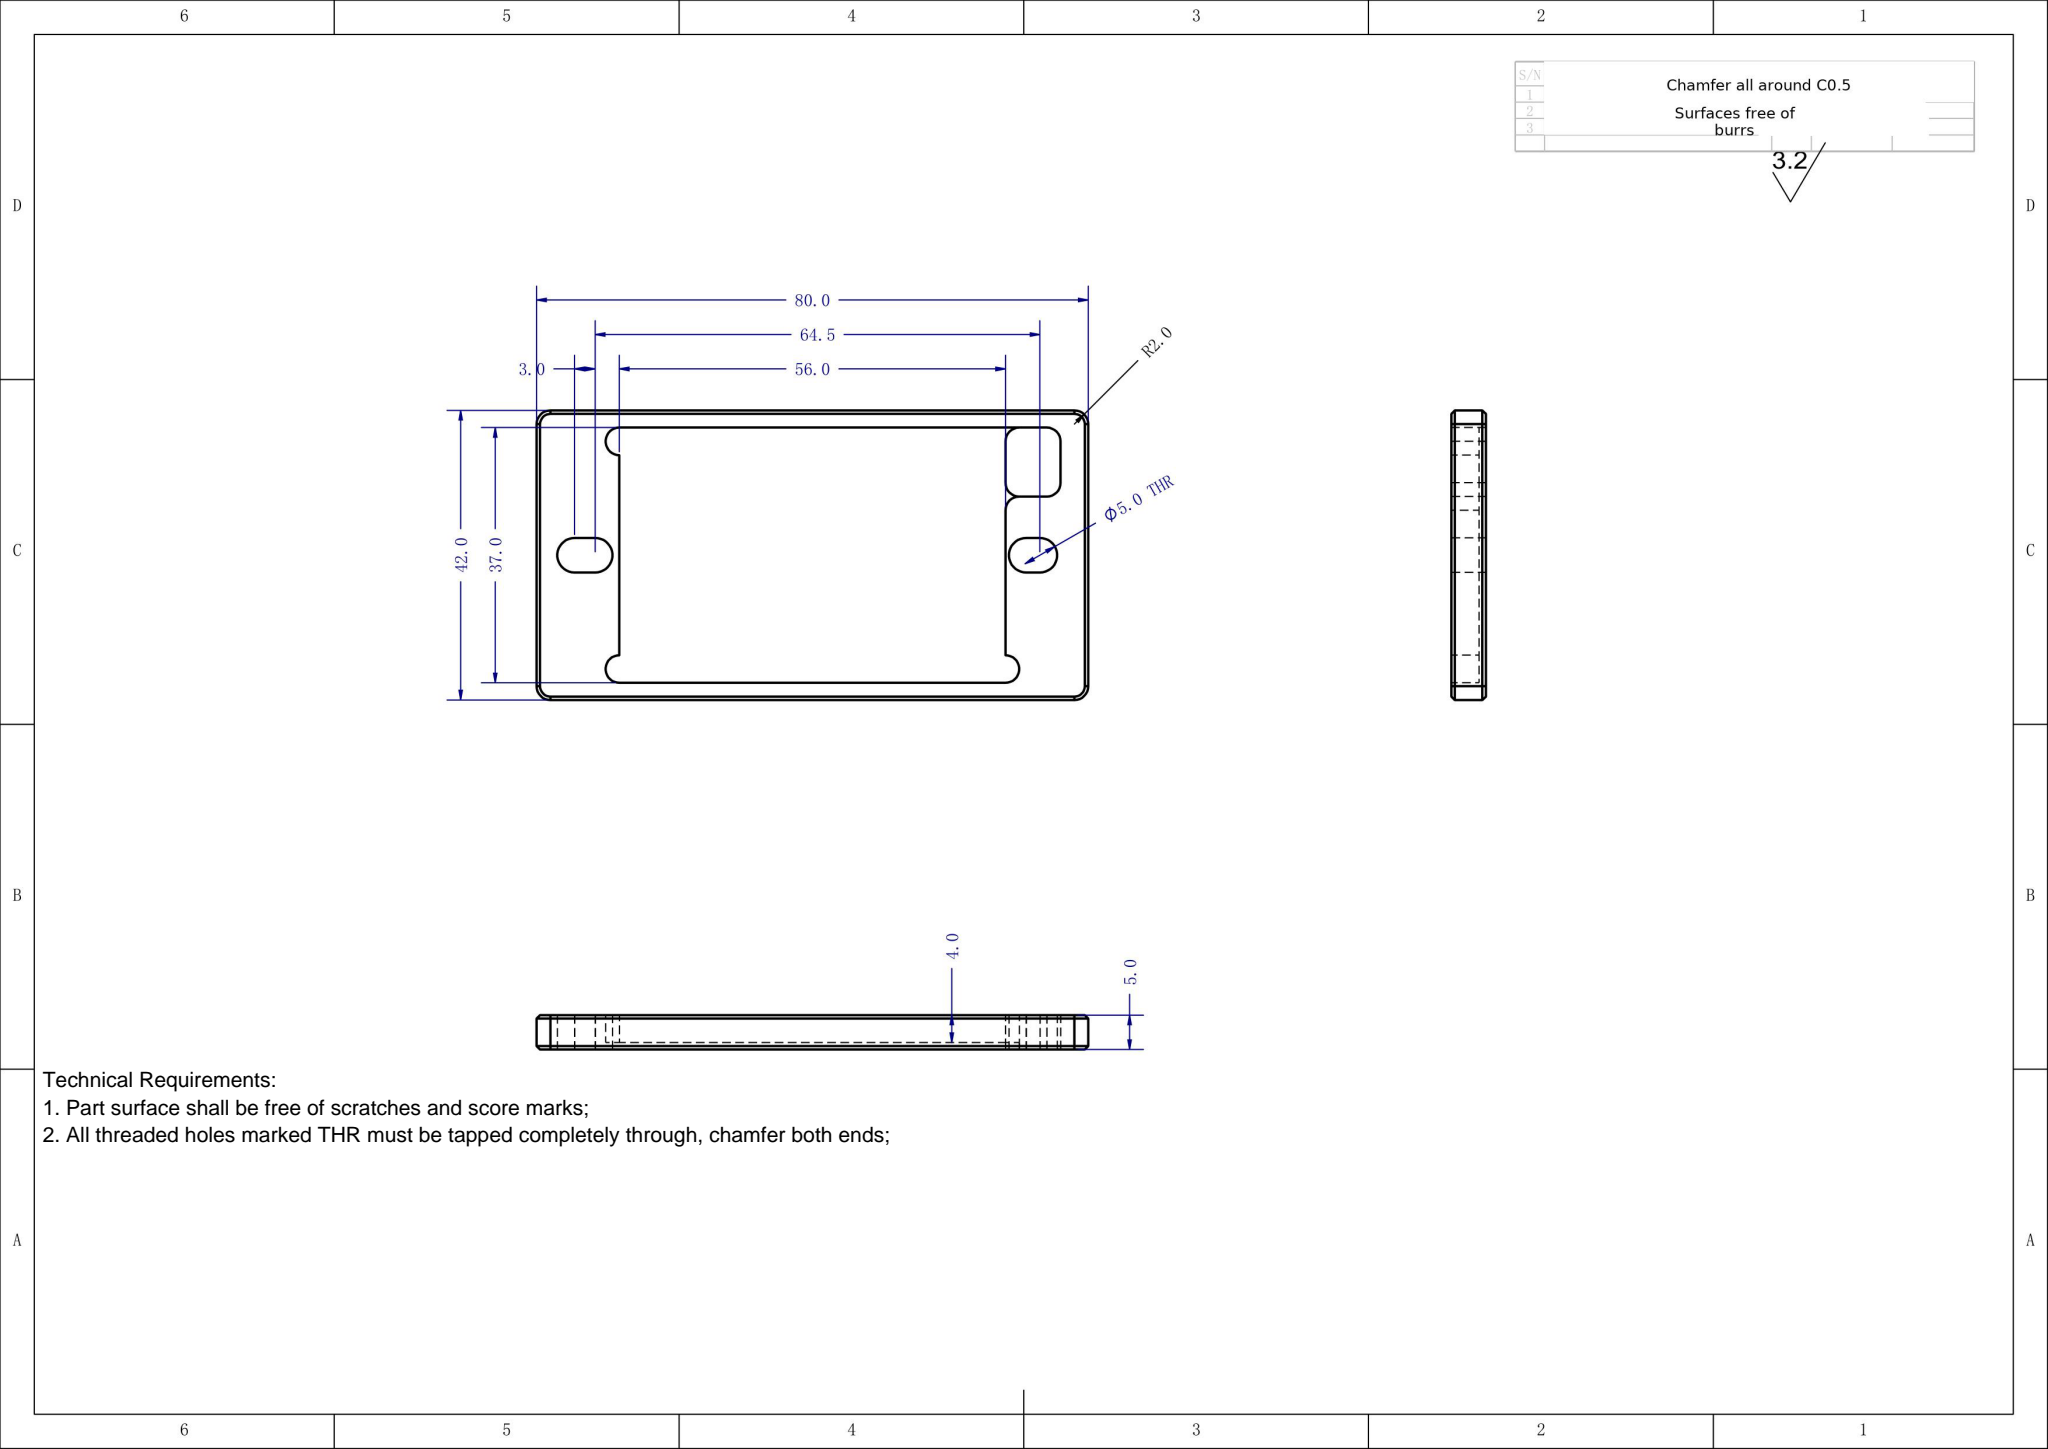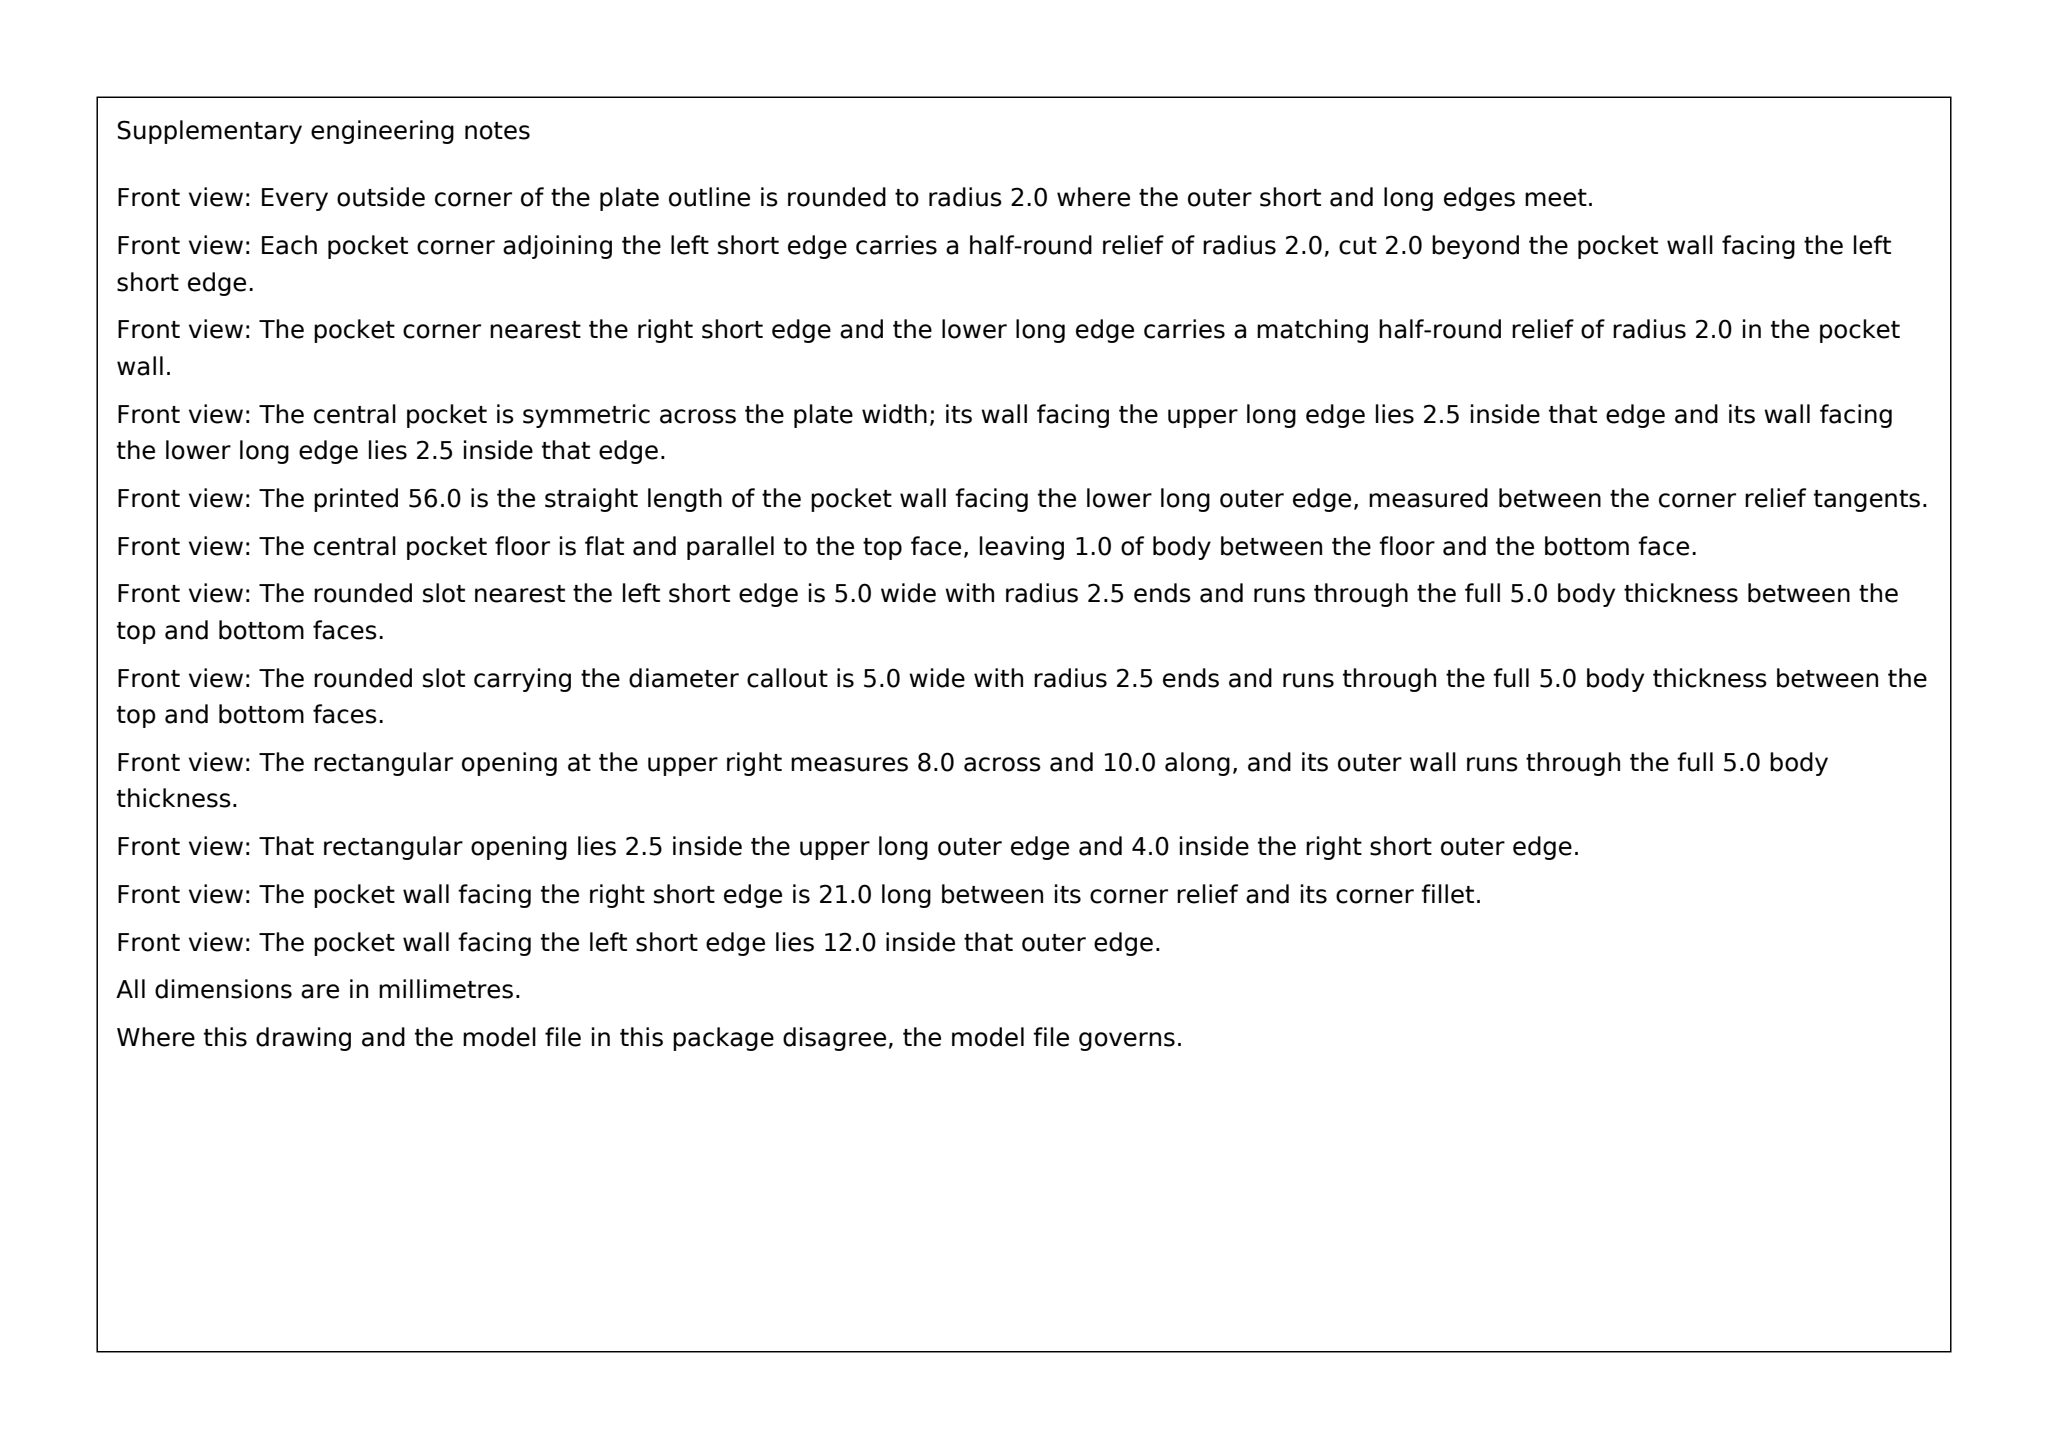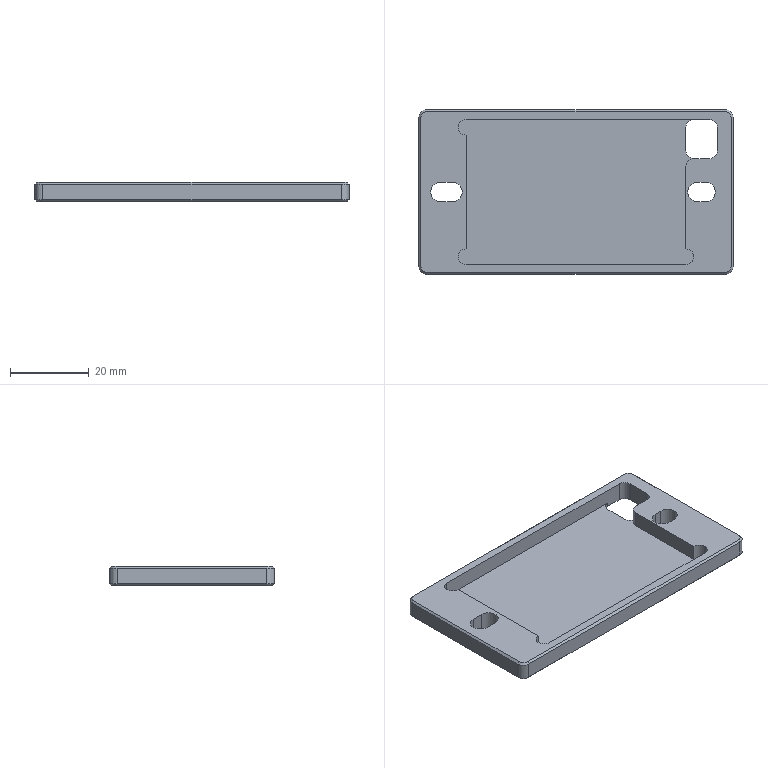Part | SolidWorks | mm | 1 solid | 53 faces | box 80 x 42 x 5 mm | volume 7645 mm3 | plane 26 | cylinder 19 | cone 8 | commonest cylinder face diameters 4 x13 5 x6
Drawing notes:
CENTRAL POCKET: 56.0 WIDE, WALLS 12.0 FROM EA END EDGE, DP 4.0 | from the solid: x-planes at 12.0 & 68.0 (bbox X=80), pocket floor z=1.0 of 5.0 thk
RH 10.0 X 8.0 POCKET: 4.0 FROM RH EDGE, 2.5 FROM TOP EDGE | from the solid: x-plane 76.0 (80-76=4.0), y-plane 39.5 (42-39.5=2.5)
RH 10.0 X 8.0 POCKET DP 4.0, FLOOR 1.0 ABV BTM, R2.0 CNRS | from the solid: z-planes 1.0 & 5.0; R2 fillet cyls dia4 at (70,31.5),(70,37.5),(74,31.5),(74,37.5)
RH Ø5.0 THR SLOT: CTRS 7.0 & 9.0 FROM RH EDGE, 21.0 FROM BTM | from the solid: dia5 cyls at x=71.0 & 73.0, y=21.0; bbox X=80
LH Ø5.0 THR SLOT: CTRS 5.5 & 8.5 FROM LH EDGE, 21.0 FROM BTM | from the solid: dia5 cyls at x=5.5 & 8.5, y=21.0
SLOT OAL: LH 8.0 (CTRS 3.0), RH 7.0 (CTRS 2.0), 5.0 WIDE | from the solid: dia5 end cyls 5.5/8.5 and 71.0/73.0, thru length 5.0
Ø5.0 THR HOLES: 90° CHAM TO Ø3.0 REF, BOTH ENDS, 8 PL | from the solid: cones[included_angle,ref_dia]=[90.0,3.0] x8
build123d program:
from build123d import *

# Parameters (mm, degrees)
SKETCH1_W                      = 80
SKETCH1_H                      = 42
BOSS_EXTRUDE1_DEPTH            = 2.5
CUT_EXTRUDE1_DEPTH             = 4
CUT_EXTRUDE2_REACH             = 47.453
SKETCH4_R                      = 2.5
CUT_EXTRUDE4_REACH             = 47.453
SKETCH10_W                     = 8
SKETCH10_H                     = 10
FILLET1_R                      = 2
CHAMFER2_SIZE                  = 0.5
FILLET2_R                      = 2
F_2021_3_1_DESIGN_CHANGE_DEPTH = 46.453


with BuildPart() as part:
    # Sketch1 → Boss-Extrude1 (new, symmetric)
    with BuildSketch(Plane.XY):
        Rectangle(SKETCH1_W, SKETCH1_H)
    extrude(amount=BOSS_EXTRUDE1_DEPTH, both=True)

    # Sketch2 → Cut-Extrude1 (cut)
    with BuildSketch(Plane.XY.offset(2.5)):
        with BuildLine():
            Line((-28, 18.5), (28, 18.5))
            ThreePointArc((28, 18.5), (30, 16.5), (28, 14.5))
            Line((28, 14.5), (28, -14.5))
            ThreePointArc((28, -14.5), (30, -16.5), (28, -18.5))
            Line((28, -18.5), (-28, -18.5))
            ThreePointArc((-28, -18.5), (-30, -16.5), (-28, -14.5))
            Line((-28, -14.5), (-28, 14.5))
            ThreePointArc((-28, 14.5), (-30, 16.5), (-28, 18.5))
        make_face()
    extrude(amount=-CUT_EXTRUDE1_DEPTH, mode=Mode.SUBTRACT)

    # Sketch4 → Cut-Extrude2 (cut, up to next)
    with BuildSketch(Plane(origin=(0, 0, -2.5), x_dir=(-1, 0, 0), z_dir=(0, 0, -1)), mode=Mode.PRIVATE) as cut_extrude2_sk1:
        with Locations((-33, 0)):
            Circle(SKETCH4_R)
    cut_extrude2_tool1 = extrude(cut_extrude2_sk1.sketch, amount=-CUT_EXTRUDE2_REACH, mode=Mode.PRIVATE) & part.part
    # Sketch4 → Cut-Extrude2 (cut, up to next)
    with BuildSketch(Plane(origin=(0, 0, -2.5), x_dir=(-1, 0, 0), z_dir=(0, 0, -1)), mode=Mode.PRIVATE) as cut_extrude2_sk2:
        with BuildLine():
            Line((31.5, 2.5), (34.5, 2.5))
            ThreePointArc((34.5, 2.5), (37, 0), (34.5, -2.5))
            Line((34.5, -2.5), (31.5, -2.5))
            ThreePointArc((31.5, -2.5), (29, 0), (31.5, 2.5))
        make_face()
    cut_extrude2_tool2 = extrude(cut_extrude2_sk2.sketch, amount=-CUT_EXTRUDE2_REACH, mode=Mode.PRIVATE) & part.part
    add(cut_extrude2_tool1.solids().sort_by_distance((33, 0, -2.5))[0], mode=Mode.SUBTRACT)
    add(cut_extrude2_tool2.solids().sort_by_distance((-33, 0, -2.5))[0], mode=Mode.SUBTRACT)

    # Sketch10 → Cut-Extrude4 (cut, up to next)
    with BuildSketch(Plane.XY.offset(2.5), mode=Mode.PRIVATE) as cut_extrude4_sk1:
        with Locations((32, 13.5)):
            Rectangle(SKETCH10_W, SKETCH10_H)
    cut_extrude4_tool1 = extrude(cut_extrude4_sk1.sketch, amount=-CUT_EXTRUDE4_REACH, mode=Mode.PRIVATE) & part.part
    add(cut_extrude4_tool1.solids().sort_by_distance((32, 13.5, 2.5))[0], mode=Mode.SUBTRACT)

    # Fillet1
    fillet1_edges = [part.edges().sort_by_distance(p)[0] for p in [
        (28, 8.5, -2),
        (28, 18.5, -2),
        (36, 18.5, 0),
        (36, 8.5, 0),
        (40, -21, 0),
        (-40, -21, 0),
        (-40, 21, 0),
        (40, 21, 0),
    ]]
    fillet(fillet1_edges, radius=FILLET1_R)

    # Chamfer2
    chamfer2_edges = [part.edges().sort_by_distance(p)[0] for p in [
        (-39.414, -20.414, -2.5),
        (-40, 0, -2.5),
        (-39.414, 20.414, -2.5),
        (-39.414, -20.414, 2.5),
        (-40, 0, 2.5),
        (-39.414, 20.414, 2.5),
    ]]
    chamfer(chamfer2_edges, length=CHAMFER2_SIZE)

    # Fillet2
    fillet2_edges = [part.edges().sort_by_distance(p)[0] for p in [
        (28, 8.5, 0.5),
    ]]
    fillet(fillet2_edges, radius=FILLET2_R)

    # Sketch11 → 2021.3.1 Design Change (cut, through all)
    with BuildSketch(Plane(origin=(0, 0, -2.5), x_dir=(-1, 0, 0), z_dir=(0, 0, -1))):
        with BuildLine():
            Line((-33, 2.5), (-31, 2.5))
            ThreePointArc((-31, 2.5), (-28.5, 0), (-31, -2.5))
            Line((-31, -2.5), (-33, -2.5))
            ThreePointArc((-33, -2.5), (-35.5, 0), (-33, 2.5))
        make_face()
    extrude(amount=-F_2021_3_1_DESIGN_CHANGE_DEPTH, mode=Mode.SUBTRACT)


solid = part.part